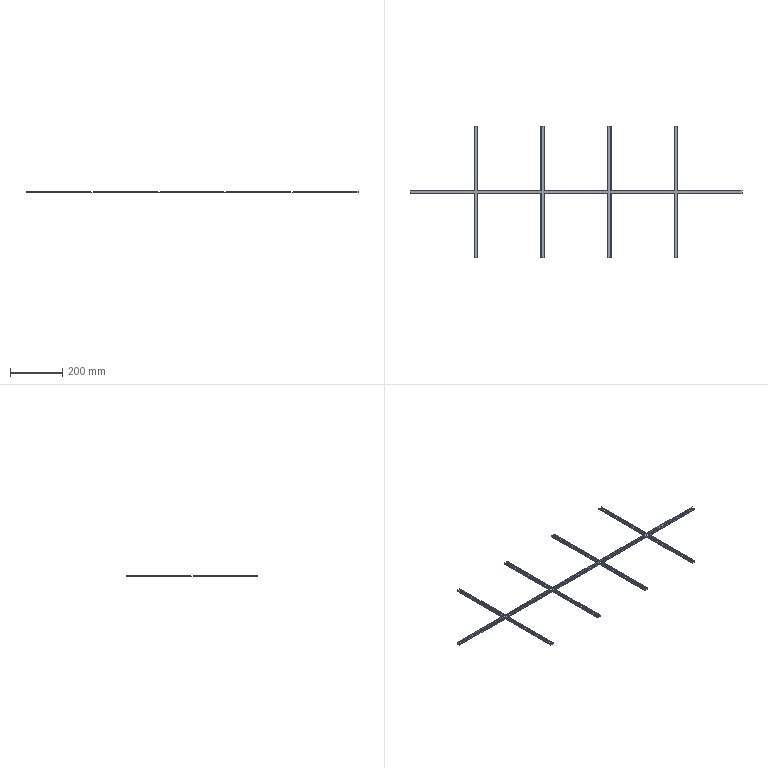Component | SolidWorks | P16BoxWeldment-1_Stiffener-1 | 1 solid | 100 faces | box 1273.5 x 505.5 x 7 mm | volume 92071 mm3 | plane 74 | cylinder 26 | commonest cylinder face diameters 3 x26
build123d program:
from build123d import *

# Parameters (mm, degrees)
BOSS_EXTRUDE1_DEPTH = 7
SHELL1_T            = -1.2
FILLET1_R           = 1.5


with BuildPart() as part:
    # Sketch1 → Boss-Extrude1 (new body)
    with BuildSketch(Plane.XY):
        Polygon((-636.75, 0), (-390.5, 0), (-390.5, -246.25), (-377.5, -246.25), (-377.5, 0), (-134.5, 0), (-134.5, -246.25), (-121.5, -246.25), (-121.5, 0), (121.5, 0), (121.5, -246.25), (134.5, -246.25), (134.5, 0), (377.5, 0), (377.5, -246.25), (390.5, -246.25), (390.5, 0), (636.75, 0), (636.75, 13), (390.5, 13), (390.5, 259.25), (377.5, 259.25), (377.5, 13), (134.5, 13), (134.5, 259.25), (121.5, 259.25), (121.5, 13), (-121.5, 13), (-121.5, 259.25), (-134.5, 259.25), (-134.5, 13), (-377.5, 13), (-377.5, 259.25), (-390.5, 259.25), (-390.5, 13), (-636.75, 13), align=None)
    extrude(amount=BOSS_EXTRUDE1_DEPTH)

    # Shell1
    shell1_openings = [part.faces().sort_by_distance(p)[0] for p in [
        (0, 6.5, 7),
        (-384, 259.25, 3.5),
        (-128, 259.25, 3.5),
        (128, 259.25, 3.5),
        (384, 259.25, 3.5),
        (636.75, 6.5, 3.5),
        (384, -246.25, 3.5),
        (128, -246.25, 3.5),
        (-128, -246.25, 3.5),
        (-384, -246.25, 3.5),
        (-636.75, 6.5, 3.5),
    ]]
    offset(amount=SHELL1_T, openings=shell1_openings, kind=Kind.INTERSECTION)

    # Fillet1
    fillet1_edges = [part.edges().sort_by_distance(p)[0] for p in [
        (-513.625, 13, 0),
        (-390.5, 136.125, 0),
        (-377.5, 136.125, 0),
        (-256, 13, 0),
        (-134.5, 136.125, 0),
        (-121.5, 136.125, 0),
        (0, 13, 0),
        (121.5, 136.125, 0),
        (134.5, 136.125, 0),
        (256, 13, 0),
        (377.5, 136.125, 0),
        (390.5, 136.125, 0),
        (513.625, 13, 0),
        (513.625, 0, 0),
        (390.5, -123.125, 0),
        (377.5, -123.125, 0),
        (256, 0, 0),
        (134.5, -123.125, 0),
        (121.5, -123.125, 0),
        (0, 0, 0),
        (-121.5, -123.125, 0),
        (-134.5, -123.125, 0),
        (-256, 0, 0),
        (-377.5, -123.125, 0),
        (-390.5, -123.125, 0),
        (-513.625, 0, 0),
    ]]
    fillet(fillet1_edges, radius=FILLET1_R)


solid = part.part

# Placed as in the assembly
solid = solid.moved(Location((-69.394, 7.042, 61.2), (0, 0, 0)))